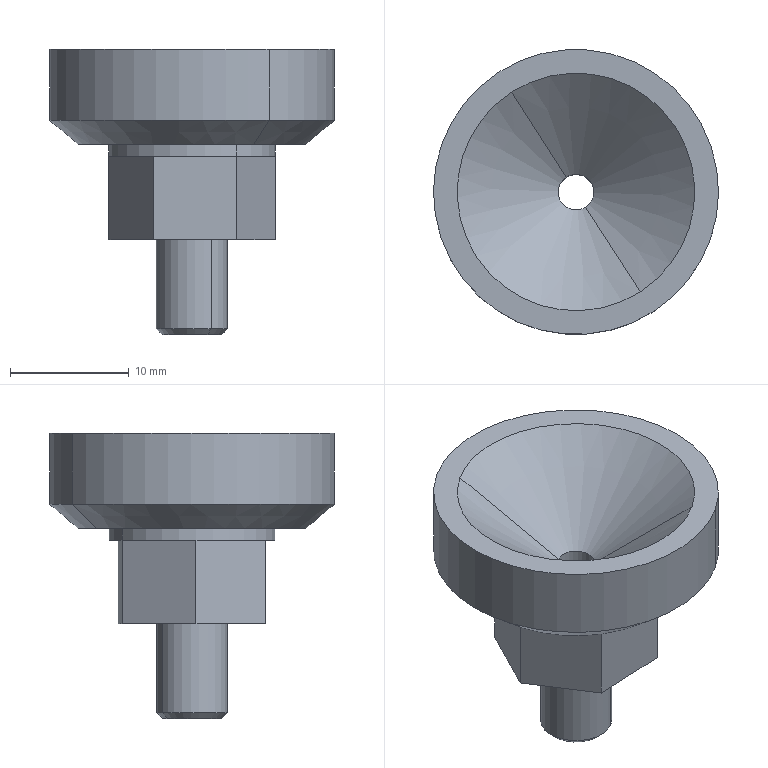Component | SolidWorks | 25-1 | 1 solid | 30 faces | box 24 x 24 x 24 mm | volume 3721 mm3 | plane 16 | cylinder 8 | cone 6 | commonest cylinder face diameters 6 x2 24 x2 3 x2 14 x2
STEP:
#1=COLOUR_RGB('',0.7922,0.8196,0.9333);
#2=FILL_AREA_STYLE_COLOUR('',#1);
#3=FILL_AREA_STYLE('',(#2));
#4=SURFACE_STYLE_FILL_AREA(#3);
#5=SURFACE_SIDE_STYLE('',(#4));
#6=SURFACE_STYLE_USAGE(.BOTH.,#5);
#7=PRESENTATION_STYLE_ASSIGNMENT((#6));
#8=CARTESIAN_POINT('',(-5.37,15.082,33.653));
#9=VERTEX_POINT('',#8);
#10=CARTESIAN_POINT('',(-5.263,14.917,33.653));
#11=VERTEX_POINT('',#10);
#12=CARTESIAN_POINT('',(-5.317,15.,33.653));
#13=DIRECTION('',(-0.,-0.,-1.));
#14=DIRECTION('',(0.541,-0.841,0.));
#15=AXIS2_PLACEMENT_3D('',#12,#13,#14);
#16=CIRCLE('',#15,0.09843);
#17=EDGE_CURVE('',#9,#11,#16,.T.);
#18=ORIENTED_EDGE('',*,*,#17,.F.);
#19=CARTESIAN_POINT('',(-5.381,15.099,33.672));
#20=VERTEX_POINT('',#19);
#21=CARTESIAN_POINT('',(-5.37,15.082,33.653));
#22=DIRECTION('',(-0.3825,0.5947,0.7071));
#23=VECTOR('',#22,39.37);
#24=LINE('',#21,#23);
#25=EDGE_CURVE('',#9,#20,#24,.T.);
#26=ORIENTED_EDGE('',*,*,#25,.T.);
#27=CARTESIAN_POINT('',(-5.253,14.9,33.672));
#28=VERTEX_POINT('',#27);
#29=CARTESIAN_POINT('',(-5.317,15.,33.672));
#30=DIRECTION('',(0.,0.,1.));
#31=DIRECTION('',(0.541,-0.841,0.));
#32=AXIS2_PLACEMENT_3D('',#29,#30,#31);
#33=CIRCLE('',#32,0.1181);
#34=EDGE_CURVE('',#28,#20,#33,.T.);
#35=ORIENTED_EDGE('',*,*,#34,.F.);
#36=CARTESIAN_POINT('',(-5.263,14.917,33.653));
#37=DIRECTION('',(0.3825,-0.5947,0.7071));
#38=VECTOR('',#37,39.37);
#39=LINE('',#36,#38);
#40=EDGE_CURVE('',#11,#28,#39,.T.);
#41=ORIENTED_EDGE('',*,*,#40,.F.);
#42=EDGE_LOOP('',(#18,#26,#35,#41));
#43=FACE_OUTER_BOUND('',#42,.T.);
#44=CARTESIAN_POINT('',(-5.317,15.,33.653));
#45=DIRECTION('',(0.,0.,1.));
#46=DIRECTION('',(0.541,-0.841,0.));
#47=AXIS2_PLACEMENT_3D('',#44,#45,#46);
#48=CONICAL_SURFACE('',#47,0.09843,0.7854);
#49=ADVANCED_FACE('',(#43),#48,.T.);
#50=CARTESIAN_POINT('',(-5.381,15.099,33.968));
#51=VERTEX_POINT('',#50);
#52=CARTESIAN_POINT('',(-5.253,14.9,33.968));
#53=VERTEX_POINT('',#52);
#54=CARTESIAN_POINT('',(-5.317,15.,33.968));
#55=DIRECTION('',(-0.,-0.,-1.));
#56=DIRECTION('',(-0.541,0.841,0.));
#57=AXIS2_PLACEMENT_3D('',#54,#55,#56);
#58=CIRCLE('',#57,0.1181);
#59=EDGE_CURVE('',#51,#53,#58,.T.);
#60=ORIENTED_EDGE('',*,*,#59,.T.);
#61=CARTESIAN_POINT('',(-5.253,14.9,33.653));
#62=DIRECTION('',(-0.,-0.,-1.));
#63=VECTOR('',#62,39.37);
#64=LINE('',#61,#63);
#65=EDGE_CURVE('',#53,#28,#64,.T.);
#66=ORIENTED_EDGE('',*,*,#65,.T.);
#67=ORIENTED_EDGE('',*,*,#34,.T.);
#68=CARTESIAN_POINT('',(-5.381,15.099,33.653));
#69=DIRECTION('',(-0.,-0.,-1.));
#70=VECTOR('',#69,39.37);
#71=LINE('',#68,#70);
#72=EDGE_CURVE('',#51,#20,#71,.T.);
#73=ORIENTED_EDGE('',*,*,#72,.F.);
#74=EDGE_LOOP('',(#60,#66,#67,#73));
#75=FACE_OUTER_BOUND('',#74,.T.);
#76=CARTESIAN_POINT('',(-5.317,15.,33.653));
#77=DIRECTION('',(-0.,-0.,-1.));
#78=DIRECTION('',(-0.541,0.841,0.));
#79=AXIS2_PLACEMENT_3D('',#76,#77,#78);
#80=CYLINDRICAL_SURFACE('',#79,0.1181);
#81=ADVANCED_FACE('',(#75),#80,.T.);
#82=CARTESIAN_POINT('',(-5.521,15.317,34.283));
#83=VERTEX_POINT('',#82);
#84=CARTESIAN_POINT('',(-5.112,14.682,34.283));
#85=VERTEX_POINT('',#84);
#86=CARTESIAN_POINT('',(-5.317,15.,34.283));
#87=DIRECTION('',(-0.,-0.,-1.));
#88=DIRECTION('',(-0.541,0.841,0.));
#89=AXIS2_PLACEMENT_3D('',#86,#87,#88);
#90=CIRCLE('',#89,0.3774);
#91=EDGE_CURVE('',#83,#85,#90,.T.);
#92=ORIENTED_EDGE('',*,*,#91,.F.);
#93=CARTESIAN_POINT('',(-5.572,15.397,34.362));
#94=VERTEX_POINT('',#93);
#95=CARTESIAN_POINT('',(-5.572,15.397,34.362));
#96=DIRECTION('',(-0.4144,0.6443,0.6428));
#97=VECTOR('',#96,39.37);
#98=LINE('',#95,#97);
#99=EDGE_CURVE('',#83,#94,#98,.T.);
#100=ORIENTED_EDGE('',*,*,#99,.T.);
#101=CARTESIAN_POINT('',(-5.061,14.602,34.362));
#102=VERTEX_POINT('',#101);
#103=CARTESIAN_POINT('',(-5.317,15.,34.362));
#104=DIRECTION('',(-0.,-0.,-1.));
#105=DIRECTION('',(-0.541,0.841,0.));
#106=AXIS2_PLACEMENT_3D('',#103,#104,#105);
#107=CIRCLE('',#106,0.4724);
#108=EDGE_CURVE('',#94,#102,#107,.T.);
#109=ORIENTED_EDGE('',*,*,#108,.T.);
#110=CARTESIAN_POINT('',(-5.061,14.602,34.362));
#111=DIRECTION('',(0.4144,-0.6443,0.6428));
#112=VECTOR('',#111,39.37);
#113=LINE('',#110,#112);
#114=EDGE_CURVE('',#85,#102,#113,.T.);
#115=ORIENTED_EDGE('',*,*,#114,.F.);
#116=EDGE_LOOP('',(#92,#100,#109,#115));
#117=FACE_OUTER_BOUND('',#116,.T.);
#118=CARTESIAN_POINT('',(-5.317,15.,34.362));
#119=DIRECTION('',(0.,0.,1.));
#120=DIRECTION('',(0.541,-0.841,0.));
#121=AXIS2_PLACEMENT_3D('',#118,#119,#120);
#122=CONICAL_SURFACE('',#121,0.4724,0.8727);
#123=ADVANCED_FACE('',(#117),#122,.T.);
#124=CARTESIAN_POINT('',(-5.572,15.397,34.598));
#125=VERTEX_POINT('',#124);
#126=CARTESIAN_POINT('',(-5.061,14.602,34.598));
#127=VERTEX_POINT('',#126);
#128=CARTESIAN_POINT('',(-5.317,15.,34.598));
#129=DIRECTION('',(-0.,-0.,-1.));
#130=DIRECTION('',(-0.541,0.841,0.));
#131=AXIS2_PLACEMENT_3D('',#128,#129,#130);
#132=CIRCLE('',#131,0.4724);
#133=EDGE_CURVE('',#125,#127,#132,.T.);
#134=ORIENTED_EDGE('',*,*,#133,.T.);
#135=CARTESIAN_POINT('',(-5.061,14.602,33.653));
#136=DIRECTION('',(-0.,-0.,-1.));
#137=VECTOR('',#136,39.37);
#138=LINE('',#135,#137);
#139=EDGE_CURVE('',#127,#102,#138,.T.);
#140=ORIENTED_EDGE('',*,*,#139,.T.);
#141=ORIENTED_EDGE('',*,*,#108,.F.);
#142=CARTESIAN_POINT('',(-5.572,15.397,33.653));
#143=DIRECTION('',(-0.,-0.,-1.));
#144=VECTOR('',#143,39.37);
#145=LINE('',#142,#144);
#146=EDGE_CURVE('',#125,#94,#145,.T.);
#147=ORIENTED_EDGE('',*,*,#146,.F.);
#148=EDGE_LOOP('',(#134,#140,#141,#147));
#149=FACE_OUTER_BOUND('',#148,.T.);
#150=CARTESIAN_POINT('',(-5.317,15.,33.653));
#151=DIRECTION('',(-0.,-0.,-1.));
#152=DIRECTION('',(-0.541,0.841,0.));
#153=AXIS2_PLACEMENT_3D('',#150,#151,#152);
#154=CYLINDRICAL_SURFACE('',#153,0.4724);
#155=ADVANCED_FACE('',(#149),#154,.T.);
#156=CARTESIAN_POINT('',(-5.285,14.95,34.317));
#157=VERTEX_POINT('',#156);
#158=CARTESIAN_POINT('',(-5.349,15.049,34.317));
#159=VERTEX_POINT('',#158);
#160=CARTESIAN_POINT('',(-5.317,15.,34.317));
#161=DIRECTION('',(-0.,-0.,-1.));
#162=DIRECTION('',(-0.541,0.841,0.));
#163=AXIS2_PLACEMENT_3D('',#160,#161,#162);
#164=CIRCLE('',#163,0.05906);
#165=EDGE_CURVE('',#157,#159,#164,.T.);
#166=ORIENTED_EDGE('',*,*,#165,.T.);
#167=CARTESIAN_POINT('',(-5.53,15.331,34.598));
#168=VERTEX_POINT('',#167);
#169=CARTESIAN_POINT('',(-5.53,15.331,34.598));
#170=DIRECTION('',(-0.4144,0.6443,0.6428));
#171=VECTOR('',#170,39.37);
#172=LINE('',#169,#171);
#173=EDGE_CURVE('',#159,#168,#172,.T.);
#174=ORIENTED_EDGE('',*,*,#173,.T.);
#175=CARTESIAN_POINT('',(-5.104,14.669,34.598));
#176=VERTEX_POINT('',#175);
#177=CARTESIAN_POINT('',(-5.317,15.,34.598));
#178=DIRECTION('',(-0.,-0.,-1.));
#179=DIRECTION('',(-0.541,0.841,0.));
#180=AXIS2_PLACEMENT_3D('',#177,#178,#179);
#181=CIRCLE('',#180,0.3937);
#182=EDGE_CURVE('',#176,#168,#181,.T.);
#183=ORIENTED_EDGE('',*,*,#182,.F.);
#184=CARTESIAN_POINT('',(-5.104,14.669,34.598));
#185=DIRECTION('',(0.4144,-0.6443,0.6428));
#186=VECTOR('',#185,39.37);
#187=LINE('',#184,#186);
#188=EDGE_CURVE('',#157,#176,#187,.T.);
#189=ORIENTED_EDGE('',*,*,#188,.F.);
#190=EDGE_LOOP('',(#166,#174,#183,#189));
#191=FACE_OUTER_BOUND('',#190,.T.);
#192=CARTESIAN_POINT('',(-5.317,15.,34.598));
#193=DIRECTION('',(0.,0.,1.));
#194=DIRECTION('',(0.541,-0.841,0.));
#195=AXIS2_PLACEMENT_3D('',#192,#193,#194);
#196=CONICAL_SURFACE('',#195,0.3937,0.8727);
#197=ADVANCED_FACE('',(#191),#196,.F.);
#198=ORIENTED_EDGE('',*,*,#165,.F.);
#199=CARTESIAN_POINT('',(-5.285,14.95,33.653));
#200=VERTEX_POINT('',#199);
#201=CARTESIAN_POINT('',(-5.285,14.95,33.653));
#202=DIRECTION('',(-0.,-0.,-1.));
#203=VECTOR('',#202,39.37);
#204=LINE('',#201,#203);
#205=EDGE_CURVE('',#157,#200,#204,.T.);
#206=ORIENTED_EDGE('',*,*,#205,.T.);
#207=CARTESIAN_POINT('',(-5.349,15.049,33.653));
#208=VERTEX_POINT('',#207);
#209=CARTESIAN_POINT('',(-5.317,15.,33.653));
#210=DIRECTION('',(-0.,-0.,-1.));
#211=DIRECTION('',(-0.541,0.841,0.));
#212=AXIS2_PLACEMENT_3D('',#209,#210,#211);
#213=CIRCLE('',#212,0.05906);
#214=EDGE_CURVE('',#200,#208,#213,.T.);
#215=ORIENTED_EDGE('',*,*,#214,.T.);
#216=CARTESIAN_POINT('',(-5.349,15.049,33.653));
#217=DIRECTION('',(-0.,-0.,-1.));
#218=VECTOR('',#217,39.37);
#219=LINE('',#216,#218);
#220=EDGE_CURVE('',#159,#208,#219,.T.);
#221=ORIENTED_EDGE('',*,*,#220,.F.);
#222=EDGE_LOOP('',(#198,#206,#215,#221));
#223=FACE_OUTER_BOUND('',#222,.T.);
#224=CARTESIAN_POINT('',(-5.317,15.,33.653));
#225=DIRECTION('',(-0.,-0.,-1.));
#226=DIRECTION('',(-0.541,0.841,0.));
#227=AXIS2_PLACEMENT_3D('',#224,#225,#226);
#228=CYLINDRICAL_SURFACE('',#227,0.05906);
#229=ADVANCED_FACE('',(#223),#228,.F.);
#230=CARTESIAN_POINT('',(-5.466,15.231,34.283));
#231=VERTEX_POINT('',#230);
#232=CARTESIAN_POINT('',(-5.168,14.768,34.283));
#233=VERTEX_POINT('',#232);
#234=CARTESIAN_POINT('',(-5.317,15.,34.283));
#235=DIRECTION('',(-0.,-0.,-1.));
#236=DIRECTION('',(-0.541,0.841,0.));
#237=AXIS2_PLACEMENT_3D('',#234,#235,#236);
#238=CIRCLE('',#237,0.2756);
#239=EDGE_CURVE('',#231,#233,#238,.T.);
#240=ORIENTED_EDGE('',*,*,#239,.T.);
#241=CARTESIAN_POINT('',(-5.168,14.768,34.243));
#242=VERTEX_POINT('',#241);
#243=CARTESIAN_POINT('',(-5.168,14.768,33.653));
#244=DIRECTION('',(-0.,-0.,-1.));
#245=VECTOR('',#244,39.37);
#246=LINE('',#243,#245);
#247=EDGE_CURVE('',#233,#242,#246,.T.);
#248=ORIENTED_EDGE('',*,*,#247,.T.);
#249=CARTESIAN_POINT('',(-5.041,15.013,34.243));
#250=VERTEX_POINT('',#249);
#251=CARTESIAN_POINT('',(-5.317,15.,34.243));
#252=DIRECTION('',(-0.,-0.,-1.));
#253=DIRECTION('',(-0.541,0.841,0.));
#254=AXIS2_PLACEMENT_3D('',#251,#252,#253);
#255=CIRCLE('',#254,0.2756);
#256=EDGE_CURVE('',#250,#242,#255,.T.);
#257=ORIENTED_EDGE('',*,*,#256,.F.);
#258=CARTESIAN_POINT('',(-5.19,15.245,34.243));
#259=VERTEX_POINT('',#258);
#260=CARTESIAN_POINT('',(-5.317,15.,34.243));
#261=DIRECTION('',(-0.,-0.,-1.));
#262=DIRECTION('',(-0.541,0.841,0.));
#263=AXIS2_PLACEMENT_3D('',#260,#261,#262);
#264=CIRCLE('',#263,0.2756);
#265=EDGE_CURVE('',#259,#250,#264,.T.);
#266=ORIENTED_EDGE('',*,*,#265,.F.);
#267=CARTESIAN_POINT('',(-5.466,15.231,34.243));
#268=VERTEX_POINT('',#267);
#269=CARTESIAN_POINT('',(-5.317,15.,34.243));
#270=DIRECTION('',(-0.,-0.,-1.));
#271=DIRECTION('',(-0.541,0.841,0.));
#272=AXIS2_PLACEMENT_3D('',#269,#270,#271);
#273=CIRCLE('',#272,0.2756);
#274=EDGE_CURVE('',#268,#259,#273,.T.);
#275=ORIENTED_EDGE('',*,*,#274,.F.);
#276=CARTESIAN_POINT('',(-5.466,15.231,33.653));
#277=DIRECTION('',(-0.,-0.,-1.));
#278=VECTOR('',#277,39.37);
#279=LINE('',#276,#278);
#280=EDGE_CURVE('',#231,#268,#279,.T.);
#281=ORIENTED_EDGE('',*,*,#280,.F.);
#282=EDGE_LOOP('',(#240,#248,#257,#266,#275,#281));
#283=FACE_OUTER_BOUND('',#282,.T.);
#284=CARTESIAN_POINT('',(-5.317,15.,33.653));
#285=DIRECTION('',(-0.,-0.,-1.));
#286=DIRECTION('',(-0.541,0.841,0.));
#287=AXIS2_PLACEMENT_3D('',#284,#285,#286);
#288=CYLINDRICAL_SURFACE('',#287,0.2756);
#289=ADVANCED_FACE('',(#283),#288,.T.);
#290=ORIENTED_EDGE('',*,*,#247,.F.);
#291=CARTESIAN_POINT('',(-5.317,15.,34.283));
#292=DIRECTION('',(-0.,-0.,-1.));
#293=DIRECTION('',(-0.541,0.841,0.));
#294=AXIS2_PLACEMENT_3D('',#291,#292,#293);
#295=CIRCLE('',#294,0.2756);
#296=EDGE_CURVE('',#233,#231,#295,.T.);
#297=ORIENTED_EDGE('',*,*,#296,.T.);
#298=ORIENTED_EDGE('',*,*,#280,.T.);
#299=CARTESIAN_POINT('',(-5.592,14.986,34.243));
#300=VERTEX_POINT('',#299);
#301=CARTESIAN_POINT('',(-5.317,15.,34.243));
#302=DIRECTION('',(-0.,-0.,-1.));
#303=DIRECTION('',(-0.541,0.841,0.));
#304=AXIS2_PLACEMENT_3D('',#301,#302,#303);
#305=CIRCLE('',#304,0.2756);
#306=EDGE_CURVE('',#300,#268,#305,.T.);
#307=ORIENTED_EDGE('',*,*,#306,.F.);
#308=CARTESIAN_POINT('',(-5.443,14.755,34.243));
#309=VERTEX_POINT('',#308);
#310=CARTESIAN_POINT('',(-5.317,15.,34.243));
#311=DIRECTION('',(-0.,-0.,-1.));
#312=DIRECTION('',(-0.541,0.841,0.));
#313=AXIS2_PLACEMENT_3D('',#310,#311,#312);
#314=CIRCLE('',#313,0.2756);
#315=EDGE_CURVE('',#309,#300,#314,.T.);
#316=ORIENTED_EDGE('',*,*,#315,.F.);
#317=CARTESIAN_POINT('',(-5.317,15.,34.243));
#318=DIRECTION('',(-0.,-0.,-1.));
#319=DIRECTION('',(-0.541,0.841,0.));
#320=AXIS2_PLACEMENT_3D('',#317,#318,#319);
#321=CIRCLE('',#320,0.2756);
#322=EDGE_CURVE('',#242,#309,#321,.T.);
#323=ORIENTED_EDGE('',*,*,#322,.F.);
#324=EDGE_LOOP('',(#290,#297,#298,#307,#316,#323));
#325=FACE_OUTER_BOUND('',#324,.T.);
#326=CARTESIAN_POINT('',(-5.317,15.,33.653));
#327=DIRECTION('',(-0.,-0.,-1.));
#328=DIRECTION('',(-0.541,0.841,0.));
#329=AXIS2_PLACEMENT_3D('',#326,#327,#328);
#330=CYLINDRICAL_SURFACE('',#329,0.2756);
#331=ADVANCED_FACE('',(#325),#330,.T.);
#332=ORIENTED_EDGE('',*,*,#59,.F.);
#333=CARTESIAN_POINT('',(-5.317,15.,33.968));
#334=DIRECTION('',(-0.,-0.,-1.));
#335=DIRECTION('',(-0.541,0.841,0.));
#336=AXIS2_PLACEMENT_3D('',#333,#334,#335);
#337=CIRCLE('',#336,0.1181);
#338=EDGE_CURVE('',#53,#51,#337,.T.);
#339=ORIENTED_EDGE('',*,*,#338,.F.);
#340=EDGE_LOOP('',(#332,#339));
#341=FACE_BOUND('',#340,.T.);
#342=CARTESIAN_POINT('',(-5.592,14.986,33.968));
#343=VERTEX_POINT('',#342);
#344=CARTESIAN_POINT('',(-5.466,15.231,33.968));
#345=VERTEX_POINT('',#344);
#346=CARTESIAN_POINT('',(-5.592,14.986,33.968));
#347=DIRECTION('',(0.4578,0.889,-0.));
#348=VECTOR('',#347,39.37);
#349=LINE('',#346,#348);
#350=EDGE_CURVE('',#343,#345,#349,.T.);
#351=ORIENTED_EDGE('',*,*,#350,.T.);
#352=CARTESIAN_POINT('',(-5.19,15.245,33.968));
#353=VERTEX_POINT('',#352);
#354=CARTESIAN_POINT('',(-5.466,15.231,33.968));
#355=DIRECTION('',(0.9988,0.04802,-0.));
#356=VECTOR('',#355,39.37);
#357=LINE('',#354,#356);
#358=EDGE_CURVE('',#345,#353,#357,.T.);
#359=ORIENTED_EDGE('',*,*,#358,.T.);
#360=CARTESIAN_POINT('',(-5.041,15.013,33.968));
#361=VERTEX_POINT('',#360);
#362=CARTESIAN_POINT('',(-5.19,15.245,33.968));
#363=DIRECTION('',(0.541,-0.841,0.));
#364=VECTOR('',#363,39.37);
#365=LINE('',#362,#364);
#366=EDGE_CURVE('',#353,#361,#365,.T.);
#367=ORIENTED_EDGE('',*,*,#366,.T.);
#368=CARTESIAN_POINT('',(-5.168,14.768,33.968));
#369=VERTEX_POINT('',#368);
#370=CARTESIAN_POINT('',(-5.041,15.013,33.968));
#371=DIRECTION('',(-0.4578,-0.889,0.));
#372=VECTOR('',#371,39.37);
#373=LINE('',#370,#372);
#374=EDGE_CURVE('',#361,#369,#373,.T.);
#375=ORIENTED_EDGE('',*,*,#374,.T.);
#376=CARTESIAN_POINT('',(-5.443,14.755,33.968));
#377=VERTEX_POINT('',#376);
#378=CARTESIAN_POINT('',(-5.168,14.768,33.968));
#379=DIRECTION('',(-0.9988,-0.04802,0.));
#380=VECTOR('',#379,39.37);
#381=LINE('',#378,#380);
#382=EDGE_CURVE('',#369,#377,#381,.T.);
#383=ORIENTED_EDGE('',*,*,#382,.T.);
#384=CARTESIAN_POINT('',(-5.443,14.755,33.968));
#385=DIRECTION('',(-0.541,0.841,-0.));
#386=VECTOR('',#385,39.37);
#387=LINE('',#384,#386);
#388=EDGE_CURVE('',#377,#343,#387,.T.);
#389=ORIENTED_EDGE('',*,*,#388,.T.);
#390=EDGE_LOOP('',(#351,#359,#367,#375,#383,#389));
#391=FACE_OUTER_BOUND('',#390,.T.);
#392=CARTESIAN_POINT('',(-5.317,15.,33.968));
#393=DIRECTION('',(0.,0.,1.));
#394=DIRECTION('',(0.541,-0.841,0.));
#395=AXIS2_PLACEMENT_3D('',#392,#393,#394);
#396=PLANE('',#395);
#397=ADVANCED_FACE('',(#341,#391),#396,.F.);
#398=ORIENTED_EDGE('',*,*,#205,.F.);
#399=CARTESIAN_POINT('',(-5.317,15.,34.317));
#400=DIRECTION('',(-0.,-0.,-1.));
#401=DIRECTION('',(-0.541,0.841,0.));
#402=AXIS2_PLACEMENT_3D('',#399,#400,#401);
#403=CIRCLE('',#402,0.05906);
#404=EDGE_CURVE('',#159,#157,#403,.T.);
#405=ORIENTED_EDGE('',*,*,#404,.F.);
#406=ORIENTED_EDGE('',*,*,#220,.T.);
#407=CARTESIAN_POINT('',(-5.317,15.,33.653));
#408=DIRECTION('',(-0.,-0.,-1.));
#409=DIRECTION('',(-0.541,0.841,0.));
#410=AXIS2_PLACEMENT_3D('',#407,#408,#409);
#411=CIRCLE('',#410,0.05906);
#412=EDGE_CURVE('',#208,#200,#411,.T.);
#413=ORIENTED_EDGE('',*,*,#412,.T.);
#414=EDGE_LOOP('',(#398,#405,#406,#413));
#415=FACE_OUTER_BOUND('',#414,.T.);
#416=CARTESIAN_POINT('',(-5.317,15.,33.653));
#417=DIRECTION('',(-0.,-0.,-1.));
#418=DIRECTION('',(-0.541,0.841,0.));
#419=AXIS2_PLACEMENT_3D('',#416,#417,#418);
#420=CYLINDRICAL_SURFACE('',#419,0.05906);
#421=ADVANCED_FACE('',(#415),#420,.F.);
#422=ORIENTED_EDGE('',*,*,#173,.F.);
#423=ORIENTED_EDGE('',*,*,#404,.T.);
#424=ORIENTED_EDGE('',*,*,#188,.T.);
#425=CARTESIAN_POINT('',(-5.317,15.,34.598));
#426=DIRECTION('',(-0.,-0.,-1.));
#427=DIRECTION('',(-0.541,0.841,0.));
#428=AXIS2_PLACEMENT_3D('',#425,#426,#427);
#429=CIRCLE('',#428,0.3937);
#430=EDGE_CURVE('',#168,#176,#429,.T.);
#431=ORIENTED_EDGE('',*,*,#430,.F.);
#432=EDGE_LOOP('',(#422,#423,#424,#431));
#433=FACE_OUTER_BOUND('',#432,.T.);
#434=CARTESIAN_POINT('',(-5.317,15.,34.598));
#435=DIRECTION('',(0.,0.,1.));
#436=DIRECTION('',(0.541,-0.841,0.));
#437=AXIS2_PLACEMENT_3D('',#434,#435,#436);
#438=CONICAL_SURFACE('',#437,0.3937,0.8727);
#439=ADVANCED_FACE('',(#433),#438,.F.);
#440=ORIENTED_EDGE('',*,*,#133,.F.);
#441=CARTESIAN_POINT('',(-5.317,15.,34.598));
#442=DIRECTION('',(-0.,-0.,-1.));
#443=DIRECTION('',(-0.541,0.841,0.));
#444=AXIS2_PLACEMENT_3D('',#441,#442,#443);
#445=CIRCLE('',#444,0.4724);
#446=EDGE_CURVE('',#127,#125,#445,.T.);
#447=ORIENTED_EDGE('',*,*,#446,.F.);
#448=EDGE_LOOP('',(#440,#447));
#449=FACE_OUTER_BOUND('',#448,.T.);
#450=ORIENTED_EDGE('',*,*,#182,.T.);
#451=ORIENTED_EDGE('',*,*,#430,.T.);
#452=EDGE_LOOP('',(#450,#451));
#453=FACE_BOUND('',#452,.T.);
#454=CARTESIAN_POINT('',(-5.317,15.,34.598));
#455=DIRECTION('',(-0.,-0.,-1.));
#456=DIRECTION('',(-0.541,0.841,-0.));
#457=AXIS2_PLACEMENT_3D('',#454,#455,#456);
#458=PLANE('',#457);
#459=ADVANCED_FACE('',(#449,#453),#458,.F.);
#460=ORIENTED_EDGE('',*,*,#139,.F.);
#461=ORIENTED_EDGE('',*,*,#446,.T.);
#462=ORIENTED_EDGE('',*,*,#146,.T.);
#463=CARTESIAN_POINT('',(-5.317,15.,34.362));
#464=DIRECTION('',(-0.,-0.,-1.));
#465=DIRECTION('',(-0.541,0.841,0.));
#466=AXIS2_PLACEMENT_3D('',#463,#464,#465);
#467=CIRCLE('',#466,0.4724);
#468=EDGE_CURVE('',#102,#94,#467,.T.);
#469=ORIENTED_EDGE('',*,*,#468,.F.);
#470=EDGE_LOOP('',(#460,#461,#462,#469));
#471=FACE_OUTER_BOUND('',#470,.T.);
#472=CARTESIAN_POINT('',(-5.317,15.,33.653));
#473=DIRECTION('',(-0.,-0.,-1.));
#474=DIRECTION('',(-0.541,0.841,0.));
#475=AXIS2_PLACEMENT_3D('',#472,#473,#474);
#476=CYLINDRICAL_SURFACE('',#475,0.4724);
#477=ADVANCED_FACE('',(#471),#476,.T.);
#478=ORIENTED_EDGE('',*,*,#99,.F.);
#479=CARTESIAN_POINT('',(-5.317,15.,34.283));
#480=DIRECTION('',(-0.,-0.,-1.));
#481=DIRECTION('',(-0.541,0.841,0.));
#482=AXIS2_PLACEMENT_3D('',#479,#480,#481);
#483=CIRCLE('',#482,0.3774);
#484=EDGE_CURVE('',#85,#83,#483,.T.);
#485=ORIENTED_EDGE('',*,*,#484,.F.);
#486=ORIENTED_EDGE('',*,*,#114,.T.);
#487=ORIENTED_EDGE('',*,*,#468,.T.);
#488=EDGE_LOOP('',(#478,#485,#486,#487));
#489=FACE_OUTER_BOUND('',#488,.T.);
#490=CARTESIAN_POINT('',(-5.317,15.,34.362));
#491=DIRECTION('',(0.,0.,1.));
#492=DIRECTION('',(0.541,-0.841,0.));
#493=AXIS2_PLACEMENT_3D('',#490,#491,#492);
#494=CONICAL_SURFACE('',#493,0.4724,0.8727);
#495=ADVANCED_FACE('',(#489),#494,.T.);
#496=ORIENTED_EDGE('',*,*,#239,.F.);
#497=ORIENTED_EDGE('',*,*,#296,.F.);
#498=EDGE_LOOP('',(#496,#497));
#499=FACE_BOUND('',#498,.T.);
#500=ORIENTED_EDGE('',*,*,#484,.T.);
#501=ORIENTED_EDGE('',*,*,#91,.T.);
#502=EDGE_LOOP('',(#500,#501));
#503=FACE_OUTER_BOUND('',#502,.T.);
#504=CARTESIAN_POINT('',(-5.317,15.,34.283));
#505=DIRECTION('',(0.,0.,1.));
#506=DIRECTION('',(0.541,-0.841,0.));
#507=AXIS2_PLACEMENT_3D('',#504,#505,#506);
#508=PLANE('',#507);
#509=ADVANCED_FACE('',(#499,#503),#508,.F.);
#510=ORIENTED_EDGE('',*,*,#65,.F.);
#511=ORIENTED_EDGE('',*,*,#338,.T.);
#512=ORIENTED_EDGE('',*,*,#72,.T.);
#513=CARTESIAN_POINT('',(-5.317,15.,33.672));
#514=DIRECTION('',(0.,0.,1.));
#515=DIRECTION('',(0.541,-0.841,0.));
#516=AXIS2_PLACEMENT_3D('',#513,#514,#515);
#517=CIRCLE('',#516,0.1181);
#518=EDGE_CURVE('',#20,#28,#517,.T.);
#519=ORIENTED_EDGE('',*,*,#518,.T.);
#520=EDGE_LOOP('',(#510,#511,#512,#519));
#521=FACE_OUTER_BOUND('',#520,.T.);
#522=CARTESIAN_POINT('',(-5.317,15.,33.653));
#523=DIRECTION('',(-0.,-0.,-1.));
#524=DIRECTION('',(-0.541,0.841,0.));
#525=AXIS2_PLACEMENT_3D('',#522,#523,#524);
#526=CYLINDRICAL_SURFACE('',#525,0.1181);
#527=ADVANCED_FACE('',(#521),#526,.T.);
#528=CARTESIAN_POINT('',(-5.317,15.,33.653));
#529=DIRECTION('',(-0.,-0.,-1.));
#530=DIRECTION('',(0.541,-0.841,0.));
#531=AXIS2_PLACEMENT_3D('',#528,#529,#530);
#532=CIRCLE('',#531,0.09843);
#533=EDGE_CURVE('',#11,#9,#532,.T.);
#534=ORIENTED_EDGE('',*,*,#533,.T.);
#535=ORIENTED_EDGE('',*,*,#17,.T.);
#536=EDGE_LOOP('',(#534,#535));
#537=FACE_OUTER_BOUND('',#536,.T.);
#538=ORIENTED_EDGE('',*,*,#412,.F.);
#539=ORIENTED_EDGE('',*,*,#214,.F.);
#540=EDGE_LOOP('',(#538,#539));
#541=FACE_BOUND('',#540,.T.);
#542=CARTESIAN_POINT('',(-5.317,15.,33.653));
#543=DIRECTION('',(0.,0.,1.));
#544=DIRECTION('',(0.541,-0.841,0.));
#545=AXIS2_PLACEMENT_3D('',#542,#543,#544);
#546=PLANE('',#545);
#547=ADVANCED_FACE('',(#537,#541),#546,.F.);
#548=ORIENTED_EDGE('',*,*,#25,.F.);
#549=ORIENTED_EDGE('',*,*,#533,.F.);
#550=ORIENTED_EDGE('',*,*,#40,.T.);
#551=ORIENTED_EDGE('',*,*,#518,.F.);
#552=EDGE_LOOP('',(#548,#549,#550,#551));
#553=FACE_OUTER_BOUND('',#552,.T.);
#554=CARTESIAN_POINT('',(-5.317,15.,33.653));
#555=DIRECTION('',(0.,0.,1.));
#556=DIRECTION('',(0.541,-0.841,0.));
#557=AXIS2_PLACEMENT_3D('',#554,#555,#556);
#558=CONICAL_SURFACE('',#557,0.09843,0.7854);
#559=ADVANCED_FACE('',(#553),#558,.T.);
#560=ORIENTED_EDGE('',*,*,#274,.T.);
#561=CARTESIAN_POINT('',(-5.466,15.231,34.243));
#562=DIRECTION('',(0.9988,0.04802,-0.));
#563=VECTOR('',#562,39.37);
#564=LINE('',#561,#563);
#565=EDGE_CURVE('',#268,#259,#564,.T.);
#566=ORIENTED_EDGE('',*,*,#565,.F.);
#567=EDGE_LOOP('',(#560,#566));
#568=FACE_OUTER_BOUND('',#567,.T.);
#569=CARTESIAN_POINT('',(-5.317,15.,34.243));
#570=DIRECTION('',(-0.,-0.,-1.));
#571=DIRECTION('',(-0.541,0.841,-0.));
#572=AXIS2_PLACEMENT_3D('',#569,#570,#571);
#573=PLANE('',#572);
#574=ADVANCED_FACE('',(#568),#573,.T.);
#575=ORIENTED_EDGE('',*,*,#265,.T.);
#576=CARTESIAN_POINT('',(-5.19,15.245,34.243));
#577=DIRECTION('',(0.541,-0.841,0.));
#578=VECTOR('',#577,39.37);
#579=LINE('',#576,#578);
#580=EDGE_CURVE('',#259,#250,#579,.T.);
#581=ORIENTED_EDGE('',*,*,#580,.F.);
#582=EDGE_LOOP('',(#575,#581));
#583=FACE_OUTER_BOUND('',#582,.T.);
#584=CARTESIAN_POINT('',(-5.317,15.,34.243));
#585=DIRECTION('',(-0.,-0.,-1.));
#586=DIRECTION('',(-0.541,0.841,-0.));
#587=AXIS2_PLACEMENT_3D('',#584,#585,#586);
#588=PLANE('',#587);
#589=ADVANCED_FACE('',(#583),#588,.T.);
#590=ORIENTED_EDGE('',*,*,#256,.T.);
#591=CARTESIAN_POINT('',(-5.041,15.013,34.243));
#592=DIRECTION('',(-0.4578,-0.889,0.));
#593=VECTOR('',#592,39.37);
#594=LINE('',#591,#593);
#595=EDGE_CURVE('',#250,#242,#594,.T.);
#596=ORIENTED_EDGE('',*,*,#595,.F.);
#597=EDGE_LOOP('',(#590,#596));
#598=FACE_OUTER_BOUND('',#597,.T.);
#599=CARTESIAN_POINT('',(-5.317,15.,34.243));
#600=DIRECTION('',(-0.,-0.,-1.));
#601=DIRECTION('',(-0.541,0.841,-0.));
#602=AXIS2_PLACEMENT_3D('',#599,#600,#601);
#603=PLANE('',#602);
#604=ADVANCED_FACE('',(#598),#603,.T.);
#605=ORIENTED_EDGE('',*,*,#322,.T.);
#606=CARTESIAN_POINT('',(-5.168,14.768,34.243));
#607=DIRECTION('',(-0.9988,-0.04802,0.));
#608=VECTOR('',#607,39.37);
#609=LINE('',#606,#608);
#610=EDGE_CURVE('',#242,#309,#609,.T.);
#611=ORIENTED_EDGE('',*,*,#610,.F.);
#612=EDGE_LOOP('',(#605,#611));
#613=FACE_OUTER_BOUND('',#612,.T.);
#614=CARTESIAN_POINT('',(-5.317,15.,34.243));
#615=DIRECTION('',(-0.,-0.,-1.));
#616=DIRECTION('',(-0.541,0.841,-0.));
#617=AXIS2_PLACEMENT_3D('',#614,#615,#616);
#618=PLANE('',#617);
#619=ADVANCED_FACE('',(#613),#618,.T.);
#620=ORIENTED_EDGE('',*,*,#315,.T.);
#621=CARTESIAN_POINT('',(-5.443,14.755,34.243));
#622=DIRECTION('',(-0.541,0.841,-0.));
#623=VECTOR('',#622,39.37);
#624=LINE('',#621,#623);
#625=EDGE_CURVE('',#309,#300,#624,.T.);
#626=ORIENTED_EDGE('',*,*,#625,.F.);
#627=EDGE_LOOP('',(#620,#626));
#628=FACE_OUTER_BOUND('',#627,.T.);
#629=CARTESIAN_POINT('',(-5.317,15.,34.243));
#630=DIRECTION('',(-0.,-0.,-1.));
#631=DIRECTION('',(-0.541,0.841,-0.));
#632=AXIS2_PLACEMENT_3D('',#629,#630,#631);
#633=PLANE('',#632);
#634=ADVANCED_FACE('',(#628),#633,.T.);
#635=ORIENTED_EDGE('',*,*,#306,.T.);
#636=CARTESIAN_POINT('',(-5.592,14.986,34.243));
#637=DIRECTION('',(0.4578,0.889,-0.));
#638=VECTOR('',#637,39.37);
#639=LINE('',#636,#638);
#640=EDGE_CURVE('',#300,#268,#639,.T.);
#641=ORIENTED_EDGE('',*,*,#640,.F.);
#642=EDGE_LOOP('',(#635,#641));
#643=FACE_OUTER_BOUND('',#642,.T.);
#644=CARTESIAN_POINT('',(-5.317,15.,34.243));
#645=DIRECTION('',(-0.,-0.,-1.));
#646=DIRECTION('',(-0.541,0.841,-0.));
#647=AXIS2_PLACEMENT_3D('',#644,#645,#646);
#648=PLANE('',#647);
#649=ADVANCED_FACE('',(#643),#648,.T.);
#650=ORIENTED_EDGE('',*,*,#350,.F.);
#651=CARTESIAN_POINT('',(-5.592,14.986,34.243));
#652=DIRECTION('',(-0.,-0.,-1.));
#653=VECTOR('',#652,39.37);
#654=LINE('',#651,#653);
#655=EDGE_CURVE('',#300,#343,#654,.T.);
#656=ORIENTED_EDGE('',*,*,#655,.F.);
#657=ORIENTED_EDGE('',*,*,#640,.T.);
#658=CARTESIAN_POINT('',(-5.466,15.231,34.243));
#659=DIRECTION('',(-0.,-0.,-1.));
#660=VECTOR('',#659,39.37);
#661=LINE('',#658,#660);
#662=EDGE_CURVE('',#268,#345,#661,.T.);
#663=ORIENTED_EDGE('',*,*,#662,.T.);
#664=EDGE_LOOP('',(#650,#656,#657,#663));
#665=FACE_OUTER_BOUND('',#664,.T.);
#666=CARTESIAN_POINT('',(-5.592,14.986,34.243));
#667=DIRECTION('',(-0.889,0.4578,-0.));
#668=DIRECTION('',(-0.4578,-0.889,0.));
#669=AXIS2_PLACEMENT_3D('',#666,#667,#668);
#670=PLANE('',#669);
#671=ADVANCED_FACE('',(#665),#670,.T.);
#672=ORIENTED_EDGE('',*,*,#388,.F.);
#673=CARTESIAN_POINT('',(-5.443,14.755,34.243));
#674=DIRECTION('',(-0.,-0.,-1.));
#675=VECTOR('',#674,39.37);
#676=LINE('',#673,#675);
#677=EDGE_CURVE('',#309,#377,#676,.T.);
#678=ORIENTED_EDGE('',*,*,#677,.F.);
#679=ORIENTED_EDGE('',*,*,#625,.T.);
#680=ORIENTED_EDGE('',*,*,#655,.T.);
#681=EDGE_LOOP('',(#672,#678,#679,#680));
#682=FACE_OUTER_BOUND('',#681,.T.);
#683=CARTESIAN_POINT('',(-5.443,14.755,34.243));
#684=DIRECTION('',(-0.841,-0.541,0.));
#685=DIRECTION('',(0.541,-0.841,0.));
#686=AXIS2_PLACEMENT_3D('',#683,#684,#685);
#687=PLANE('',#686);
#688=ADVANCED_FACE('',(#682),#687,.T.);
#689=ORIENTED_EDGE('',*,*,#382,.F.);
#690=CARTESIAN_POINT('',(-5.168,14.768,34.243));
#691=DIRECTION('',(-0.,-0.,-1.));
#692=VECTOR('',#691,39.37);
#693=LINE('',#690,#692);
#694=EDGE_CURVE('',#242,#369,#693,.T.);
#695=ORIENTED_EDGE('',*,*,#694,.F.);
#696=ORIENTED_EDGE('',*,*,#610,.T.);
#697=ORIENTED_EDGE('',*,*,#677,.T.);
#698=EDGE_LOOP('',(#689,#695,#696,#697));
#699=FACE_OUTER_BOUND('',#698,.T.);
#700=CARTESIAN_POINT('',(-5.168,14.768,34.243));
#701=DIRECTION('',(0.04802,-0.9988,0.));
#702=DIRECTION('',(0.9988,0.04802,-0.));
#703=AXIS2_PLACEMENT_3D('',#700,#701,#702);
#704=PLANE('',#703);
#705=ADVANCED_FACE('',(#699),#704,.T.);
#706=ORIENTED_EDGE('',*,*,#374,.F.);
#707=CARTESIAN_POINT('',(-5.041,15.013,34.243));
#708=DIRECTION('',(-0.,-0.,-1.));
#709=VECTOR('',#708,39.37);
#710=LINE('',#707,#709);
#711=EDGE_CURVE('',#250,#361,#710,.T.);
#712=ORIENTED_EDGE('',*,*,#711,.F.);
#713=ORIENTED_EDGE('',*,*,#595,.T.);
#714=ORIENTED_EDGE('',*,*,#694,.T.);
#715=EDGE_LOOP('',(#706,#712,#713,#714));
#716=FACE_OUTER_BOUND('',#715,.T.);
#717=CARTESIAN_POINT('',(-5.041,15.013,34.243));
#718=DIRECTION('',(0.889,-0.4578,0.));
#719=DIRECTION('',(0.4578,0.889,-0.));
#720=AXIS2_PLACEMENT_3D('',#717,#718,#719);
#721=PLANE('',#720);
#722=ADVANCED_FACE('',(#716),#721,.T.);
#723=ORIENTED_EDGE('',*,*,#366,.F.);
#724=CARTESIAN_POINT('',(-5.19,15.245,34.243));
#725=DIRECTION('',(-0.,-0.,-1.));
#726=VECTOR('',#725,39.37);
#727=LINE('',#724,#726);
#728=EDGE_CURVE('',#259,#353,#727,.T.);
#729=ORIENTED_EDGE('',*,*,#728,.F.);
#730=ORIENTED_EDGE('',*,*,#580,.T.);
#731=ORIENTED_EDGE('',*,*,#711,.T.);
#732=EDGE_LOOP('',(#723,#729,#730,#731));
#733=FACE_OUTER_BOUND('',#732,.T.);
#734=CARTESIAN_POINT('',(-5.19,15.245,34.243));
#735=DIRECTION('',(0.841,0.541,-0.));
#736=DIRECTION('',(-0.541,0.841,-0.));
#737=AXIS2_PLACEMENT_3D('',#734,#735,#736);
#738=PLANE('',#737);
#739=ADVANCED_FACE('',(#733),#738,.T.);
#740=ORIENTED_EDGE('',*,*,#358,.F.);
#741=ORIENTED_EDGE('',*,*,#662,.F.);
#742=ORIENTED_EDGE('',*,*,#565,.T.);
#743=ORIENTED_EDGE('',*,*,#728,.T.);
#744=EDGE_LOOP('',(#740,#741,#742,#743));
#745=FACE_OUTER_BOUND('',#744,.T.);
#746=CARTESIAN_POINT('',(-5.466,15.231,34.243));
#747=DIRECTION('',(-0.04802,0.9988,-0.));
#748=DIRECTION('',(-0.9988,-0.04802,0.));
#749=AXIS2_PLACEMENT_3D('',#746,#747,#748);
#750=PLANE('',#749);
#751=ADVANCED_FACE('',(#745),#750,.T.);
#752=CLOSED_SHELL('',(#49,#81,#123,#155,#197,#229,#289,#331,#397,#421,#439,#459,#477,#495,#509,#527,#547,#559,#574,#589,#604,#619,#634,#649,#671,#688,#705,#722,#739,#751));
#753=MANIFOLD_SOLID_BREP('',#752);
#754=STYLED_ITEM('',(#7),#753);
#755=PRESENTATION_LAYER_ASSIGNMENT('','',(#754));
#756=CARTESIAN_POINT('',(0.,0.,0.));
#757=DIRECTION('',(0.,0.,1.));
#758=DIRECTION('',(1.,0.,0.));
#759=AXIS2_PLACEMENT_3D('',#756,#757,#758);
#760=(LENGTH_UNIT()NAMED_UNIT(*)SI_UNIT($,.METRE.));
#761=LENGTH_MEASURE_WITH_UNIT(LENGTH_MEASURE(0.0254),#760);
#762=DIMENSIONAL_EXPONENTS(1.,0.,0.,0.,0.,0.,0.);
#763=(CONVERSION_BASED_UNIT('',#761)LENGTH_UNIT()NAMED_UNIT(#762));
#764=UNCERTAINTY_MEASURE_WITH_UNIT(LENGTH_MEASURE(0.00001),#763,'','');
#765=(NAMED_UNIT(*)PLANE_ANGLE_UNIT()SI_UNIT($,.RADIAN.));
#766=(NAMED_UNIT(*)SI_UNIT($,.STERADIAN.)SOLID_ANGLE_UNIT());
#767=(GEOMETRIC_REPRESENTATION_CONTEXT(3)GLOBAL_UNCERTAINTY_ASSIGNED_CONTEXT((#764))GLOBAL_UNIT_ASSIGNED_CONTEXT((#763,#765,#766))REPRESENTATION_CONTEXT('',''));
#768=ADVANCED_BREP_SHAPE_REPRESENTATION('',(#753,#759),#767);
#769=(LENGTH_UNIT()NAMED_UNIT(*)SI_UNIT($,.METRE.));
#770=LENGTH_MEASURE_WITH_UNIT(LENGTH_MEASURE(0.0254),#769);
#771=DIMENSIONAL_EXPONENTS(1.,0.,0.,0.,0.,0.,0.);
#772=(CONVERSION_BASED_UNIT('',#770)LENGTH_UNIT()NAMED_UNIT(#771));
#773=UNCERTAINTY_MEASURE_WITH_UNIT(LENGTH_MEASURE(0.00001),#772,'','');
#774=(NAMED_UNIT(*)PLANE_ANGLE_UNIT()SI_UNIT($,.RADIAN.));
#775=(NAMED_UNIT(*)SI_UNIT($,.STERADIAN.)SOLID_ANGLE_UNIT());
#776=(GEOMETRIC_REPRESENTATION_CONTEXT(3)GLOBAL_UNCERTAINTY_ASSIGNED_CONTEXT((#773))GLOBAL_UNIT_ASSIGNED_CONTEXT((#772,#774,#775))REPRESENTATION_CONTEXT('',''));
#777=MECHANICAL_DESIGN_GEOMETRIC_PRESENTATION_REPRESENTATION('',(#754),#776);